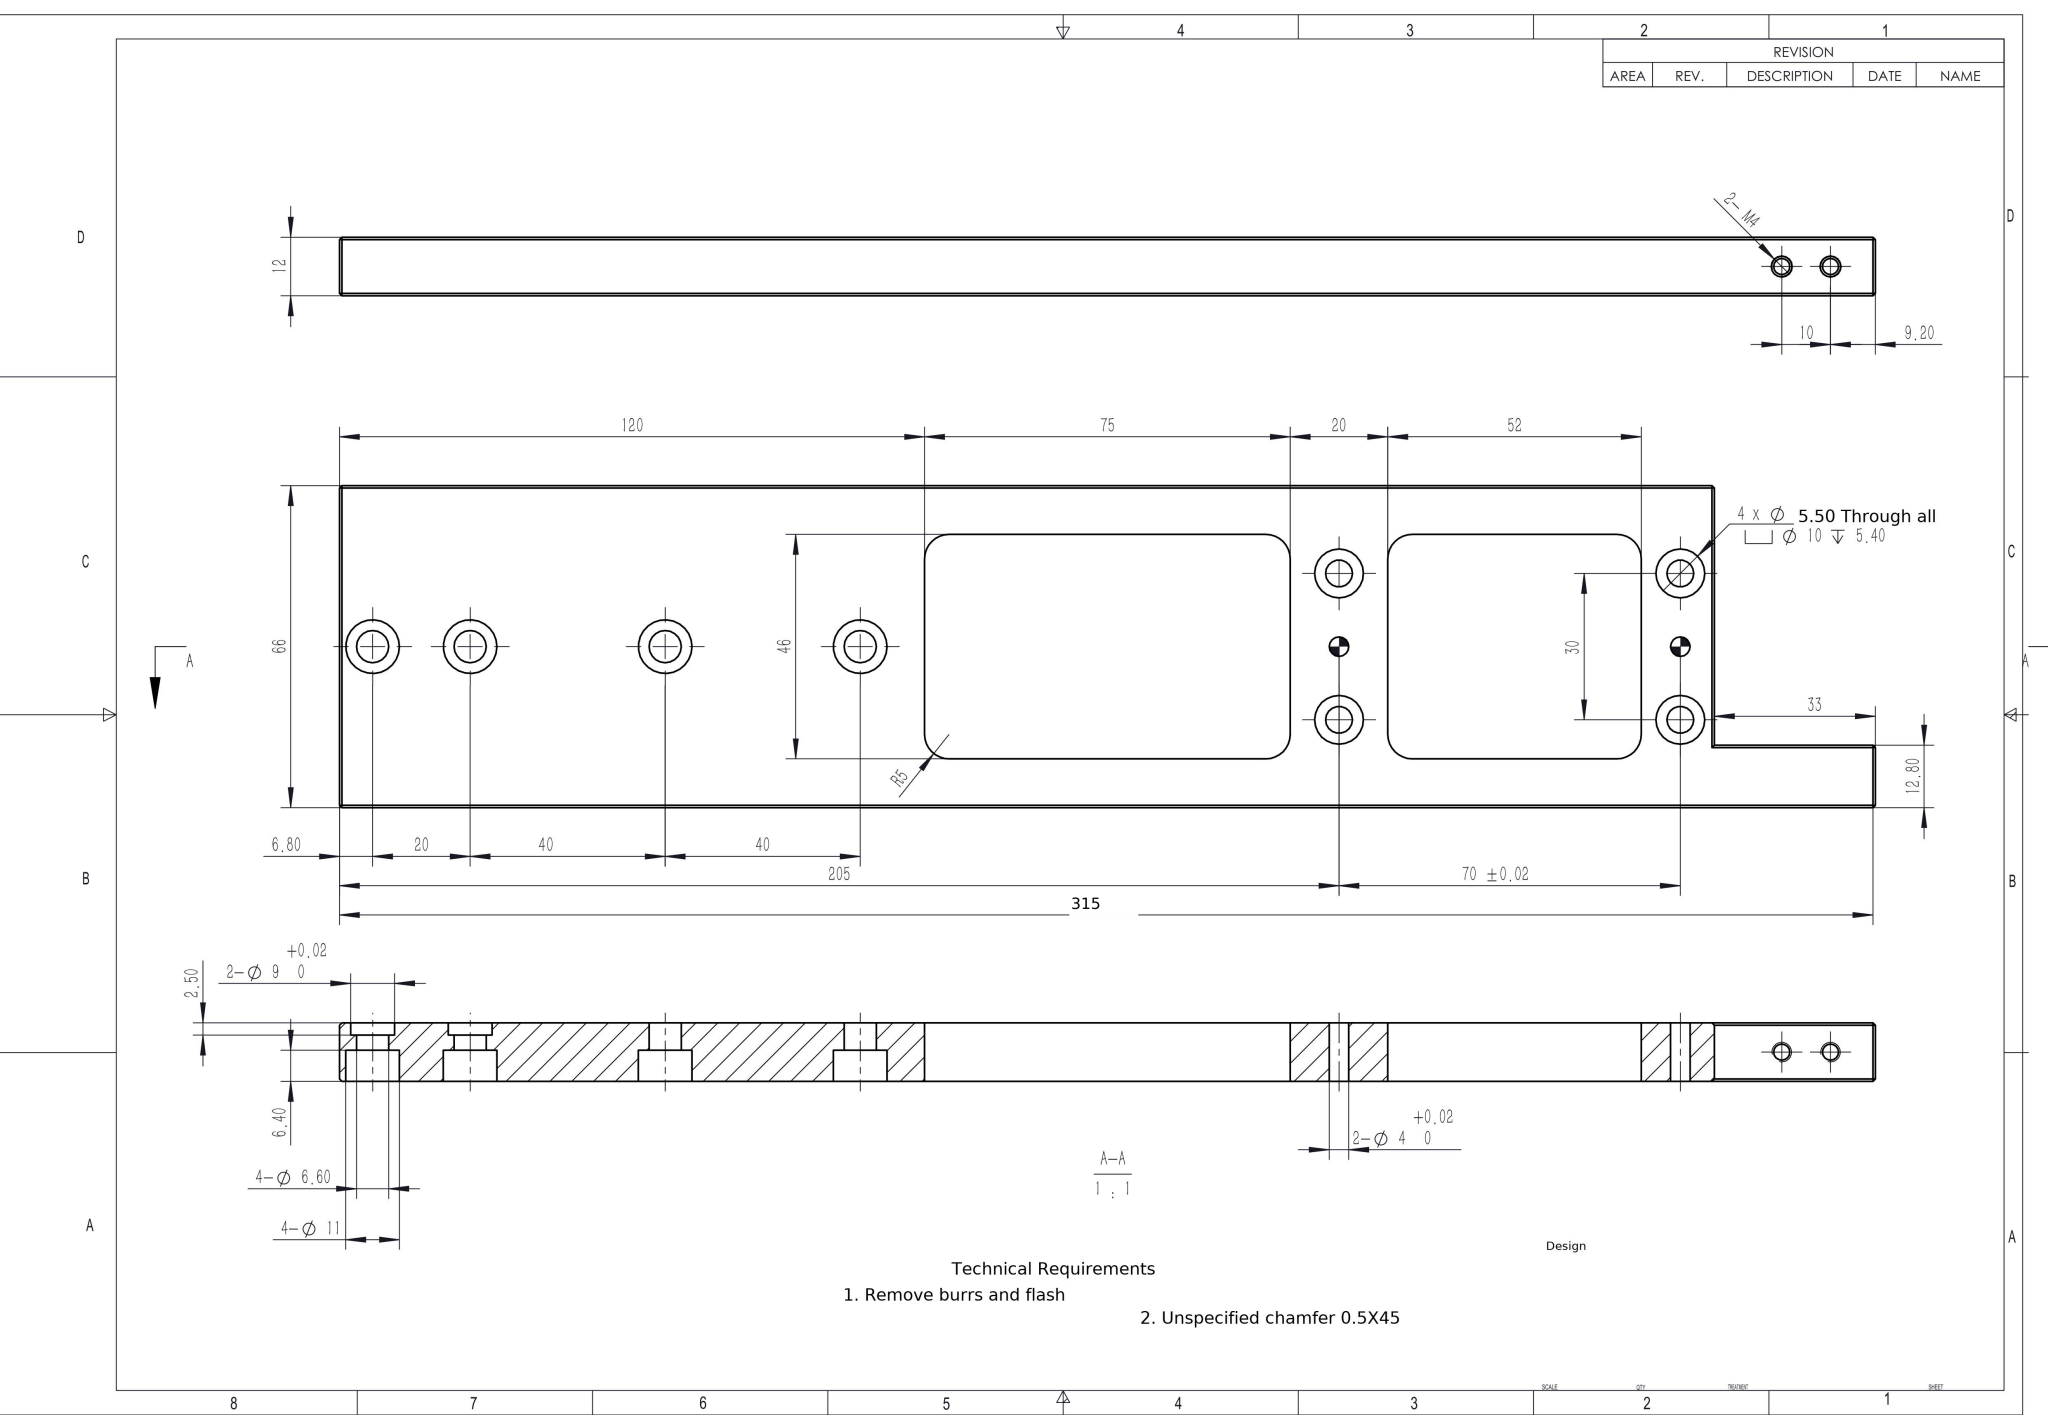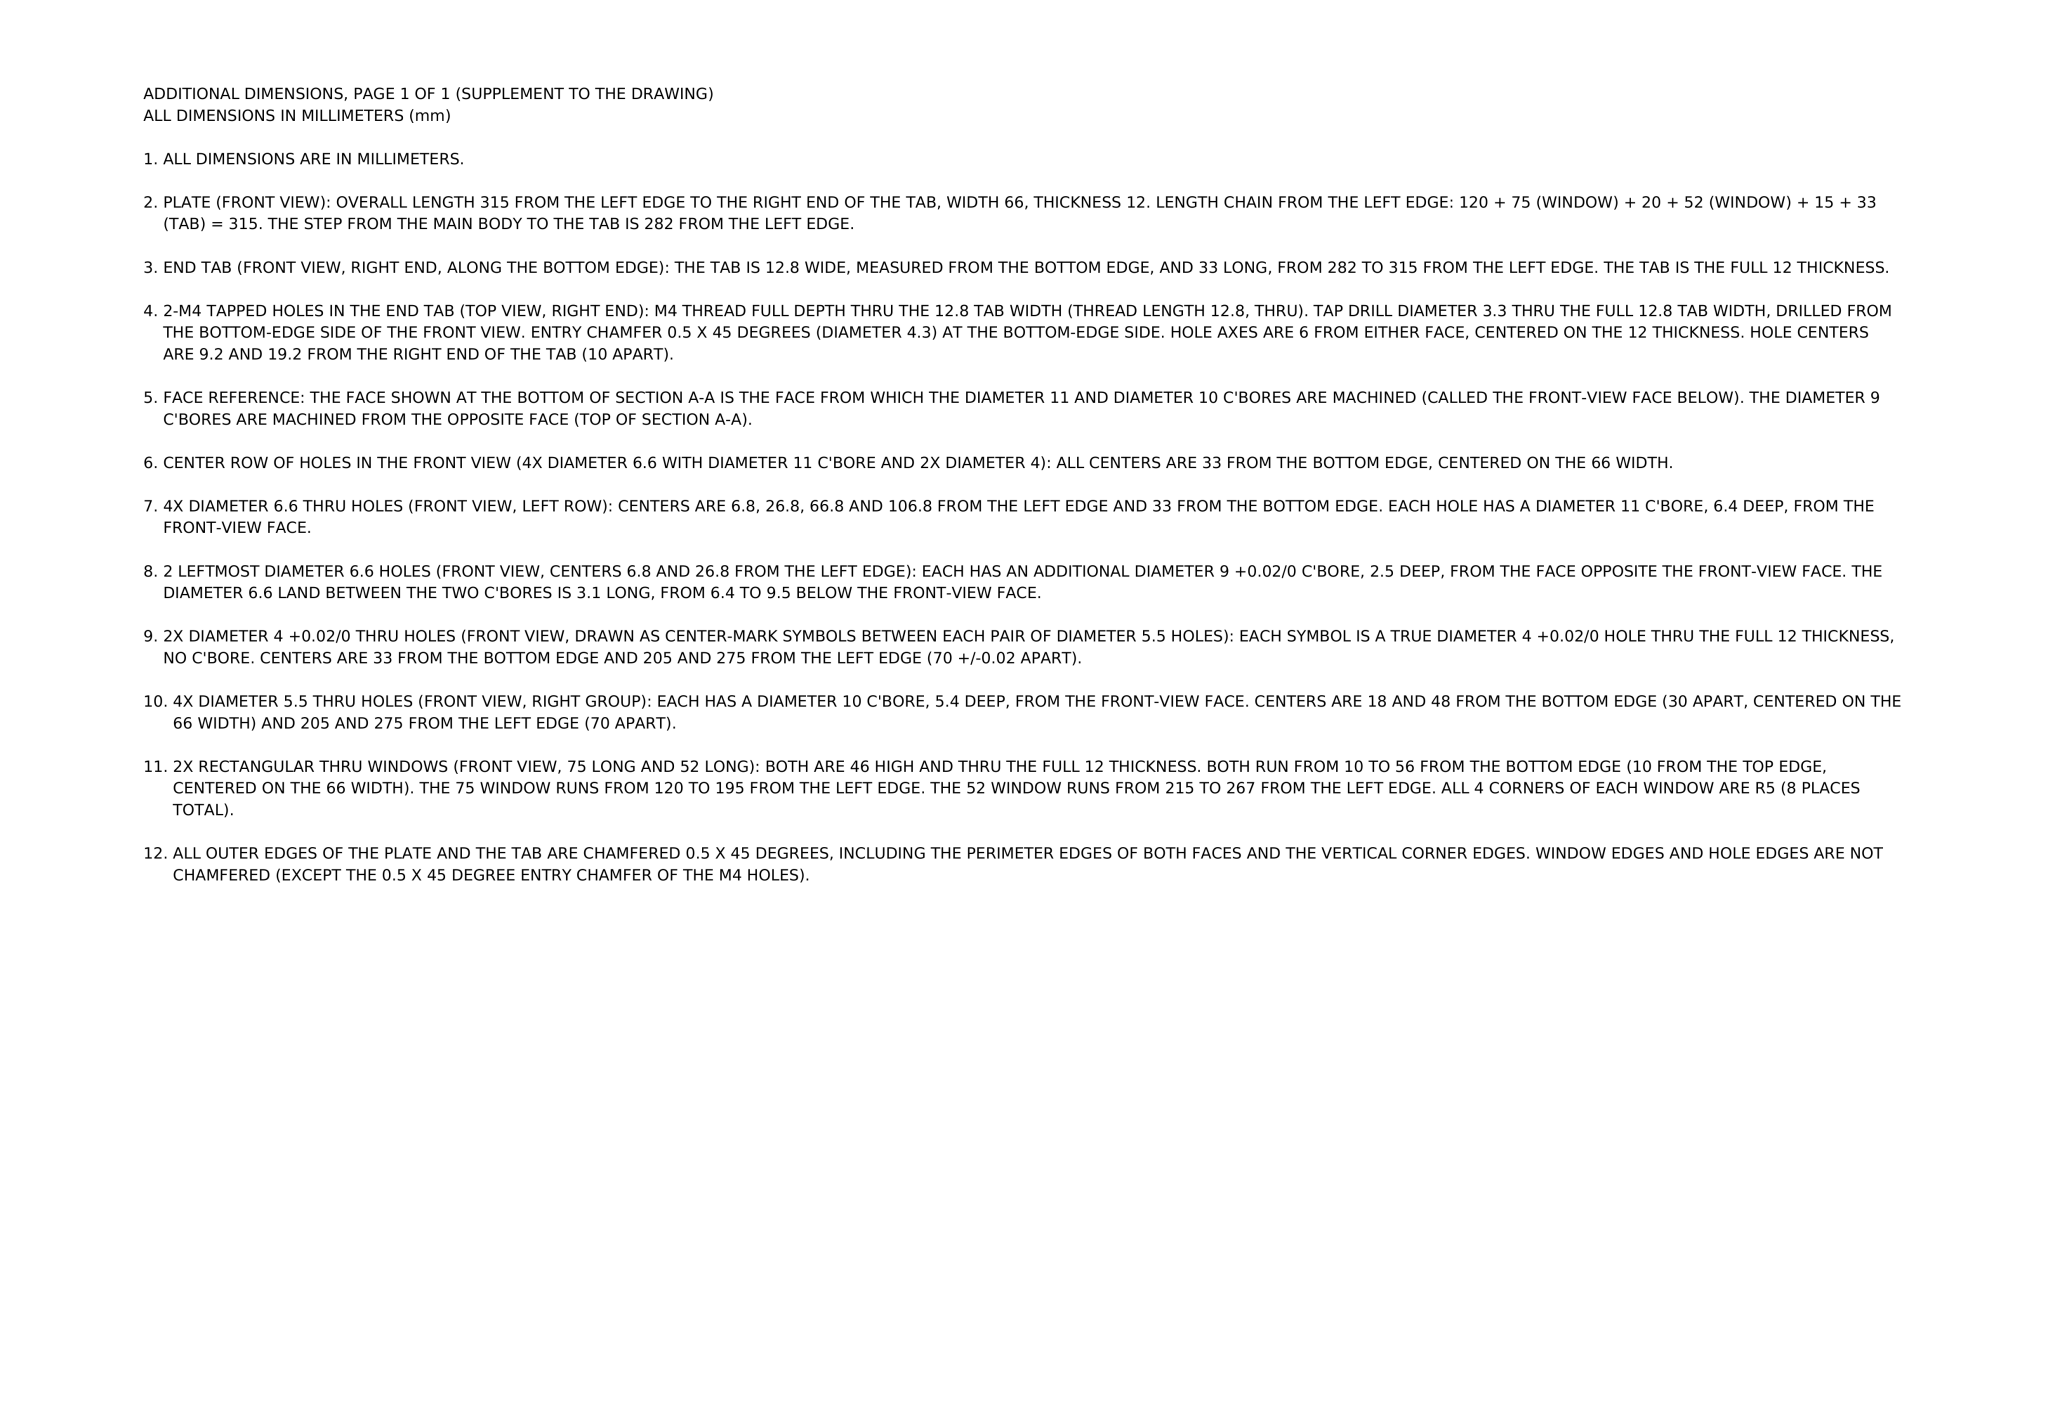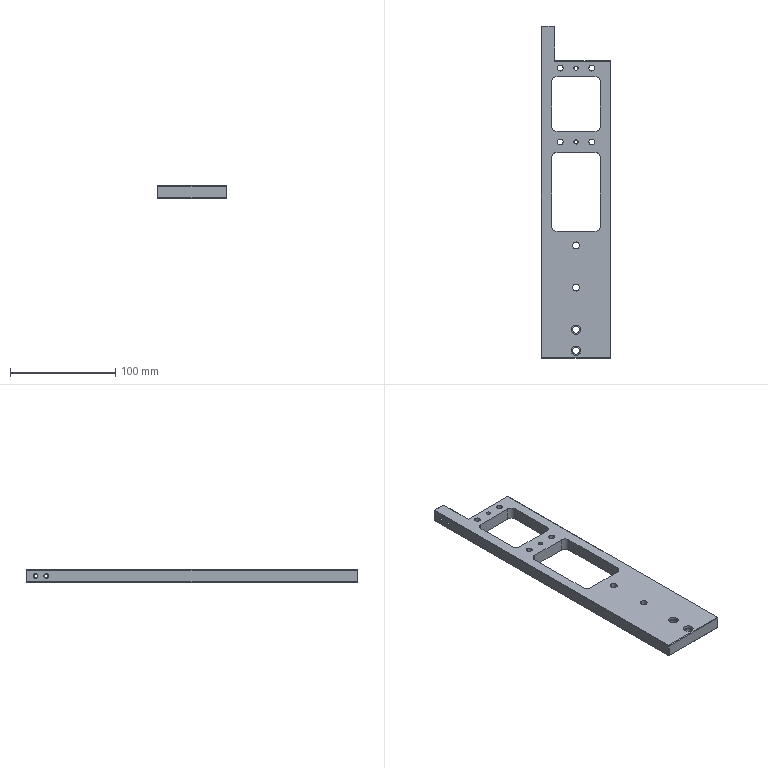Part | NX | mm | 1 solid | 109 faces | box 66 x 315 x 12 mm | volume 152433 mm3 | plane 53 | cylinder 52 | cone 4 | commonest cylinder face diameters 10 x16 11 x8 6.6 x8 5.5 x8 9 x4 4 x4 3.3 x4